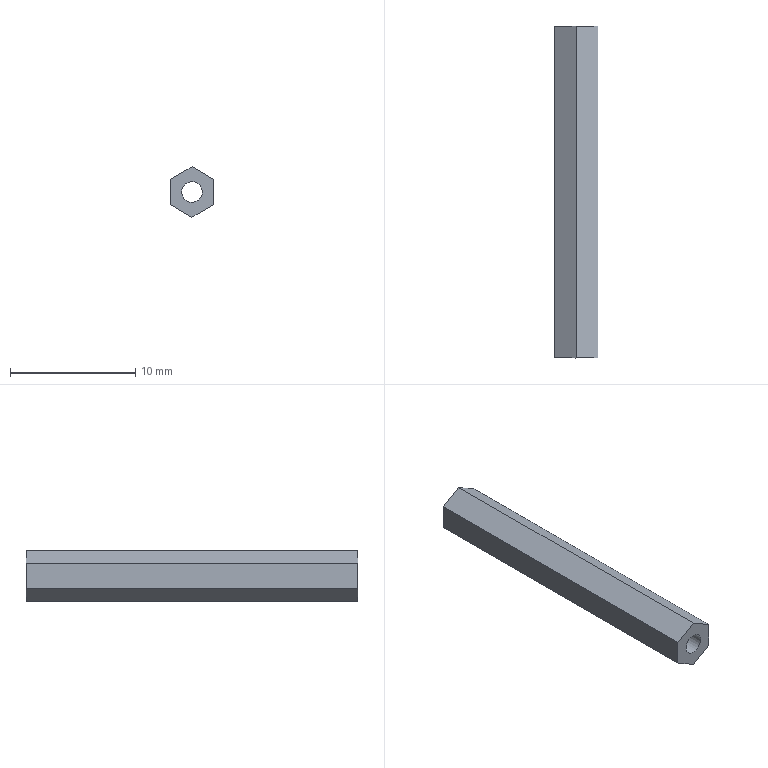Component | NX | 12 | 1 solid | 9 faces | box 3.51 x 26.5 x 4.04 mm | volume 224 mm3 | plane 8 | cylinder 1 | commonest cylinder face diameters 1.65 x1
STEP:
#1=CARTESIAN_POINT('',(0.,0.,0.));
#2=DIRECTION('',(0.,0.,1.));
#3=DIRECTION('',(1.,0.,0.));
#4=AXIS2_PLACEMENT_3D('',#1,#2,#3);
#5=CARTESIAN_POINT('',(-341.815,190.749,-163.207));
#6=VERTEX_POINT('',#5);
#7=CARTESIAN_POINT('',(-341.815,164.249,-163.207));
#8=VERTEX_POINT('',#7);
#9=CARTESIAN_POINT('',(-341.815,164.249,-163.207));
#10=DIRECTION('',(0.,-1.,0.));
#11=VECTOR('',#10,1.);
#12=LINE('',#9,#11);
#13=CARTESIAN_POINT('',(-340.071,164.249,-164.228));
#14=DIRECTION('',(-0.5052,0.,-0.863));
#15=DIRECTION('',(-0.863,0.,0.5052));
#16=AXIS2_PLACEMENT_3D('',#13,#14,#15);
#17=PLANE('',#16);
#18=CARTESIAN_POINT('',(2.021,0.));
#19=DIRECTION('',(0.,-1.));
#20=VECTOR('',#19,1.);
#21=LINE('',#18,#20);
#22=(GEOMETRIC_REPRESENTATION_CONTEXT(2)PARAMETRIC_REPRESENTATION_CONTEXT()REPRESENTATION_CONTEXT('',''));
#23=DEFINITIONAL_REPRESENTATION('',(#21),#22);
#24=PCURVE('',#17,#23);
#25=CARTESIAN_POINT('',(-341.815,164.249,-163.207));
#26=DIRECTION('',(0.4948,0.,-0.869));
#27=DIRECTION('',(0.,-1.,0.));
#28=AXIS2_PLACEMENT_3D('',#25,#26,#27);
#29=PLANE('',#28);
#30=CARTESIAN_POINT('',(0.,0.));
#31=DIRECTION('',(1.,0.));
#32=VECTOR('',#31,1.);
#33=LINE('',#30,#32);
#34=(GEOMETRIC_REPRESENTATION_CONTEXT(2)PARAMETRIC_REPRESENTATION_CONTEXT()REPRESENTATION_CONTEXT('',''));
#35=DEFINITIONAL_REPRESENTATION('',(#33),#34);
#36=PCURVE('',#29,#35);
#37=SURFACE_CURVE('',#12,(#24,#36),.PCURVE_S1.);
#38=EDGE_CURVE('',#6,#8,#37,.T.);
#39=ORIENTED_EDGE('',*,*,#38,.T.);
#40=CARTESIAN_POINT('',(-340.071,164.249,-164.228));
#41=VERTEX_POINT('',#40);
#42=CARTESIAN_POINT('',(-340.071,164.249,-164.228));
#43=DIRECTION('',(-0.863,0.,0.5052));
#44=VECTOR('',#43,1.);
#45=LINE('',#42,#44);
#46=CARTESIAN_POINT('',(0.,0.));
#47=DIRECTION('',(1.,0.));
#48=VECTOR('',#47,1.);
#49=LINE('',#46,#48);
#50=(GEOMETRIC_REPRESENTATION_CONTEXT(2)PARAMETRIC_REPRESENTATION_CONTEXT()REPRESENTATION_CONTEXT('',''));
#51=DEFINITIONAL_REPRESENTATION('',(#49),#50);
#52=PCURVE('',#17,#51);
#53=CARTESIAN_POINT('',(-341.827,164.249,-165.227));
#54=DIRECTION('',(0.,-1.,0.));
#55=DIRECTION('',(-0.869,0.,-0.4948));
#56=AXIS2_PLACEMENT_3D('',#53,#54,#55);
#57=PLANE('',#56);
#58=CARTESIAN_POINT('',(-2.021,-0.));
#59=DIRECTION('',(0.5,-0.866));
#60=VECTOR('',#59,1.);
#61=LINE('',#58,#60);
#62=(GEOMETRIC_REPRESENTATION_CONTEXT(2)PARAMETRIC_REPRESENTATION_CONTEXT()REPRESENTATION_CONTEXT('',''));
#63=DEFINITIONAL_REPRESENTATION('',(#61),#62);
#64=PCURVE('',#57,#63);
#65=SURFACE_CURVE('',#45,(#52,#64),.PCURVE_S1.);
#66=EDGE_CURVE('',#41,#8,#65,.T.);
#67=ORIENTED_EDGE('',*,*,#66,.F.);
#68=CARTESIAN_POINT('',(-340.071,190.749,-164.228));
#69=VERTEX_POINT('',#68);
#70=CARTESIAN_POINT('',(-340.071,164.249,-164.228));
#71=DIRECTION('',(0.,1.,0.));
#72=VECTOR('',#71,1.);
#73=LINE('',#70,#72);
#74=CARTESIAN_POINT('',(0.,0.));
#75=DIRECTION('',(0.,1.));
#76=VECTOR('',#75,1.);
#77=LINE('',#74,#76);
#78=(GEOMETRIC_REPRESENTATION_CONTEXT(2)PARAMETRIC_REPRESENTATION_CONTEXT()REPRESENTATION_CONTEXT('',''));
#79=DEFINITIONAL_REPRESENTATION('',(#77),#78);
#80=PCURVE('',#17,#79);
#81=CARTESIAN_POINT('',(-340.083,164.249,-166.248));
#82=DIRECTION('',(-1.,0.,0.005967));
#83=DIRECTION('',(0.005967,0.,1.));
#84=AXIS2_PLACEMENT_3D('',#81,#82,#83);
#85=PLANE('',#84);
#86=CARTESIAN_POINT('',(2.021,0.));
#87=DIRECTION('',(0.,1.));
#88=VECTOR('',#87,1.);
#89=LINE('',#86,#88);
#90=(GEOMETRIC_REPRESENTATION_CONTEXT(2)PARAMETRIC_REPRESENTATION_CONTEXT()REPRESENTATION_CONTEXT('',''));
#91=DEFINITIONAL_REPRESENTATION('',(#89),#90);
#92=PCURVE('',#85,#91);
#93=SURFACE_CURVE('',#73,(#80,#92),.PCURVE_S1.);
#94=EDGE_CURVE('',#41,#69,#93,.T.);
#95=ORIENTED_EDGE('',*,*,#94,.T.);
#96=CARTESIAN_POINT('',(-340.071,190.749,-164.228));
#97=DIRECTION('',(-0.863,0.,0.5052));
#98=VECTOR('',#97,1.);
#99=LINE('',#96,#98);
#100=CARTESIAN_POINT('',(0.,26.5));
#101=DIRECTION('',(1.,0.));
#102=VECTOR('',#101,1.);
#103=LINE('',#100,#102);
#104=(GEOMETRIC_REPRESENTATION_CONTEXT(2)PARAMETRIC_REPRESENTATION_CONTEXT()REPRESENTATION_CONTEXT('',''));
#105=DEFINITIONAL_REPRESENTATION('',(#103),#104);
#106=PCURVE('',#17,#105);
#107=CARTESIAN_POINT('',(-341.827,190.749,-165.227));
#108=DIRECTION('',(0.,-1.,0.));
#109=DIRECTION('',(-0.869,0.,-0.4948));
#110=AXIS2_PLACEMENT_3D('',#107,#108,#109);
#111=PLANE('',#110);
#112=CARTESIAN_POINT('',(-2.021,-0.));
#113=DIRECTION('',(0.5,-0.866));
#114=VECTOR('',#113,1.);
#115=LINE('',#112,#114);
#116=(GEOMETRIC_REPRESENTATION_CONTEXT(2)PARAMETRIC_REPRESENTATION_CONTEXT()REPRESENTATION_CONTEXT('',''));
#117=DEFINITIONAL_REPRESENTATION('',(#115),#116);
#118=PCURVE('',#111,#117);
#119=SURFACE_CURVE('',#99,(#106,#118),.PCURVE_S1.);
#120=EDGE_CURVE('',#69,#6,#119,.T.);
#121=ORIENTED_EDGE('',*,*,#120,.T.);
#122=EDGE_LOOP('',(#39,#67,#95,#121));
#123=FACE_BOUND('',#122,.T.);
#124=ADVANCED_FACE('',(#123),#17,.F.);
#125=CARTESIAN_POINT('',(-343.571,190.749,-164.207));
#126=VERTEX_POINT('',#125);
#127=CARTESIAN_POINT('',(-343.571,164.249,-164.207));
#128=VERTEX_POINT('',#127);
#129=CARTESIAN_POINT('',(-343.571,164.249,-164.207));
#130=DIRECTION('',(0.,-1.,0.));
#131=VECTOR('',#130,1.);
#132=LINE('',#129,#131);
#133=CARTESIAN_POINT('',(0.,2.021));
#134=DIRECTION('',(1.,0.));
#135=VECTOR('',#134,1.);
#136=LINE('',#133,#135);
#137=(GEOMETRIC_REPRESENTATION_CONTEXT(2)PARAMETRIC_REPRESENTATION_CONTEXT()REPRESENTATION_CONTEXT('',''));
#138=DEFINITIONAL_REPRESENTATION('',(#136),#137);
#139=PCURVE('',#29,#138);
#140=CARTESIAN_POINT('',(-343.571,164.249,-164.207));
#141=DIRECTION('',(1.,0.,-0.005967));
#142=DIRECTION('',(-0.005967,0.,-1.));
#143=AXIS2_PLACEMENT_3D('',#140,#141,#142);
#144=PLANE('',#143);
#145=CARTESIAN_POINT('',(0.,0.));
#146=DIRECTION('',(0.,-1.));
#147=VECTOR('',#146,1.);
#148=LINE('',#145,#147);
#149=(GEOMETRIC_REPRESENTATION_CONTEXT(2)PARAMETRIC_REPRESENTATION_CONTEXT()REPRESENTATION_CONTEXT('',''));
#150=DEFINITIONAL_REPRESENTATION('',(#148),#149);
#151=PCURVE('',#144,#150);
#152=SURFACE_CURVE('',#132,(#139,#151),.PCURVE_S1.);
#153=EDGE_CURVE('',#126,#128,#152,.T.);
#154=ORIENTED_EDGE('',*,*,#153,.T.);
#155=CARTESIAN_POINT('',(-342.693,164.249,-163.707));
#156=DIRECTION('',(-0.869,0.,-0.4948));
#157=VECTOR('',#156,1.);
#158=LINE('',#155,#157);
#159=CARTESIAN_POINT('',(0.,1.01));
#160=DIRECTION('',(0.,1.));
#161=VECTOR('',#160,1.);
#162=LINE('',#159,#161);
#163=(GEOMETRIC_REPRESENTATION_CONTEXT(2)PARAMETRIC_REPRESENTATION_CONTEXT()REPRESENTATION_CONTEXT('',''));
#164=DEFINITIONAL_REPRESENTATION('',(#162),#163);
#165=PCURVE('',#29,#164);
#166=CARTESIAN_POINT('',(-0.,-1.75));
#167=DIRECTION('',(1.,0.));
#168=VECTOR('',#167,1.);
#169=LINE('',#166,#168);
#170=(GEOMETRIC_REPRESENTATION_CONTEXT(2)PARAMETRIC_REPRESENTATION_CONTEXT()REPRESENTATION_CONTEXT('',''));
#171=DEFINITIONAL_REPRESENTATION('',(#169),#170);
#172=PCURVE('',#57,#171);
#173=SURFACE_CURVE('',#158,(#165,#172),.PCURVE_S1.);
#174=EDGE_CURVE('',#8,#128,#173,.T.);
#175=ORIENTED_EDGE('',*,*,#174,.F.);
#176=ORIENTED_EDGE('',*,*,#38,.F.);
#177=CARTESIAN_POINT('',(-342.693,190.749,-163.707));
#178=DIRECTION('',(-0.869,0.,-0.4948));
#179=VECTOR('',#178,1.);
#180=LINE('',#177,#179);
#181=CARTESIAN_POINT('',(-26.5,1.01));
#182=DIRECTION('',(0.,1.));
#183=VECTOR('',#182,1.);
#184=LINE('',#181,#183);
#185=(GEOMETRIC_REPRESENTATION_CONTEXT(2)PARAMETRIC_REPRESENTATION_CONTEXT()REPRESENTATION_CONTEXT('',''));
#186=DEFINITIONAL_REPRESENTATION('',(#184),#185);
#187=PCURVE('',#29,#186);
#188=CARTESIAN_POINT('',(-0.,-1.75));
#189=DIRECTION('',(1.,0.));
#190=VECTOR('',#189,1.);
#191=LINE('',#188,#190);
#192=(GEOMETRIC_REPRESENTATION_CONTEXT(2)PARAMETRIC_REPRESENTATION_CONTEXT()REPRESENTATION_CONTEXT('',''));
#193=DEFINITIONAL_REPRESENTATION('',(#191),#192);
#194=PCURVE('',#111,#193);
#195=SURFACE_CURVE('',#180,(#187,#194),.PCURVE_S1.);
#196=EDGE_CURVE('',#6,#126,#195,.T.);
#197=ORIENTED_EDGE('',*,*,#196,.T.);
#198=EDGE_LOOP('',(#154,#175,#176,#197));
#199=FACE_BOUND('',#198,.T.);
#200=ADVANCED_FACE('',(#199),#29,.F.);
#201=CARTESIAN_POINT('',(-343.583,190.749,-166.227));
#202=VERTEX_POINT('',#201);
#203=CARTESIAN_POINT('',(-343.583,164.249,-166.227));
#204=VERTEX_POINT('',#203);
#205=CARTESIAN_POINT('',(-343.583,164.249,-166.227));
#206=DIRECTION('',(0.,-1.,0.));
#207=VECTOR('',#206,1.);
#208=LINE('',#205,#207);
#209=CARTESIAN_POINT('',(2.021,0.));
#210=DIRECTION('',(0.,-1.));
#211=VECTOR('',#210,1.);
#212=LINE('',#209,#211);
#213=(GEOMETRIC_REPRESENTATION_CONTEXT(2)PARAMETRIC_REPRESENTATION_CONTEXT()REPRESENTATION_CONTEXT('',''));
#214=DEFINITIONAL_REPRESENTATION('',(#212),#213);
#215=PCURVE('',#144,#214);
#216=CARTESIAN_POINT('',(-343.583,164.249,-166.227));
#217=DIRECTION('',(0.5052,0.,0.863));
#218=DIRECTION('',(0.863,0.,-0.5052));
#219=AXIS2_PLACEMENT_3D('',#216,#217,#218);
#220=PLANE('',#219);
#221=CARTESIAN_POINT('',(0.,0.));
#222=DIRECTION('',(0.,-1.));
#223=VECTOR('',#222,1.);
#224=LINE('',#221,#223);
#225=(GEOMETRIC_REPRESENTATION_CONTEXT(2)PARAMETRIC_REPRESENTATION_CONTEXT()REPRESENTATION_CONTEXT('',''));
#226=DEFINITIONAL_REPRESENTATION('',(#224),#225);
#227=PCURVE('',#220,#226);
#228=SURFACE_CURVE('',#208,(#215,#227),.PCURVE_S1.);
#229=EDGE_CURVE('',#202,#204,#228,.T.);
#230=ORIENTED_EDGE('',*,*,#229,.T.);
#231=CARTESIAN_POINT('',(-343.571,164.249,-164.207));
#232=DIRECTION('',(-0.005967,0.,-1.));
#233=VECTOR('',#232,1.);
#234=LINE('',#231,#233);
#235=CARTESIAN_POINT('',(0.,0.));
#236=DIRECTION('',(1.,0.));
#237=VECTOR('',#236,1.);
#238=LINE('',#235,#237);
#239=(GEOMETRIC_REPRESENTATION_CONTEXT(2)PARAMETRIC_REPRESENTATION_CONTEXT()REPRESENTATION_CONTEXT('',''));
#240=DEFINITIONAL_REPRESENTATION('',(#238),#239);
#241=PCURVE('',#144,#240);
#242=CARTESIAN_POINT('',(1.01,-1.75));
#243=DIRECTION('',(0.5,0.866));
#244=VECTOR('',#243,1.);
#245=LINE('',#242,#244);
#246=(GEOMETRIC_REPRESENTATION_CONTEXT(2)PARAMETRIC_REPRESENTATION_CONTEXT()REPRESENTATION_CONTEXT('',''));
#247=DEFINITIONAL_REPRESENTATION('',(#245),#246);
#248=PCURVE('',#57,#247);
#249=SURFACE_CURVE('',#234,(#241,#248),.PCURVE_S1.);
#250=EDGE_CURVE('',#128,#204,#249,.T.);
#251=ORIENTED_EDGE('',*,*,#250,.F.);
#252=ORIENTED_EDGE('',*,*,#153,.F.);
#253=CARTESIAN_POINT('',(-343.571,190.749,-164.207));
#254=DIRECTION('',(-0.005967,0.,-1.));
#255=VECTOR('',#254,1.);
#256=LINE('',#253,#255);
#257=CARTESIAN_POINT('',(0.,26.5));
#258=DIRECTION('',(1.,0.));
#259=VECTOR('',#258,1.);
#260=LINE('',#257,#259);
#261=(GEOMETRIC_REPRESENTATION_CONTEXT(2)PARAMETRIC_REPRESENTATION_CONTEXT()REPRESENTATION_CONTEXT('',''));
#262=DEFINITIONAL_REPRESENTATION('',(#260),#261);
#263=PCURVE('',#144,#262);
#264=CARTESIAN_POINT('',(1.01,-1.75));
#265=DIRECTION('',(0.5,0.866));
#266=VECTOR('',#265,1.);
#267=LINE('',#264,#266);
#268=(GEOMETRIC_REPRESENTATION_CONTEXT(2)PARAMETRIC_REPRESENTATION_CONTEXT()REPRESENTATION_CONTEXT('',''));
#269=DEFINITIONAL_REPRESENTATION('',(#267),#268);
#270=PCURVE('',#111,#269);
#271=SURFACE_CURVE('',#256,(#263,#270),.PCURVE_S1.);
#272=EDGE_CURVE('',#126,#202,#271,.T.);
#273=ORIENTED_EDGE('',*,*,#272,.T.);
#274=EDGE_LOOP('',(#230,#251,#252,#273));
#275=FACE_BOUND('',#274,.T.);
#276=ADVANCED_FACE('',(#275),#144,.F.);
#277=CARTESIAN_POINT('',(-341.839,190.749,-167.248));
#278=VERTEX_POINT('',#277);
#279=CARTESIAN_POINT('',(-341.839,164.249,-167.248));
#280=VERTEX_POINT('',#279);
#281=CARTESIAN_POINT('',(-341.839,164.249,-167.248));
#282=DIRECTION('',(0.,-1.,0.));
#283=VECTOR('',#282,1.);
#284=LINE('',#281,#283);
#285=CARTESIAN_POINT('',(2.021,0.));
#286=DIRECTION('',(0.,-1.));
#287=VECTOR('',#286,1.);
#288=LINE('',#285,#287);
#289=(GEOMETRIC_REPRESENTATION_CONTEXT(2)PARAMETRIC_REPRESENTATION_CONTEXT()REPRESENTATION_CONTEXT('',''));
#290=DEFINITIONAL_REPRESENTATION('',(#288),#289);
#291=PCURVE('',#220,#290);
#292=CARTESIAN_POINT('',(-341.839,164.249,-167.248));
#293=DIRECTION('',(-0.4948,0.,0.869));
#294=DIRECTION('',(0.869,0.,0.4948));
#295=AXIS2_PLACEMENT_3D('',#292,#293,#294);
#296=PLANE('',#295);
#297=CARTESIAN_POINT('',(0.,0.));
#298=DIRECTION('',(0.,-1.));
#299=VECTOR('',#298,1.);
#300=LINE('',#297,#299);
#301=(GEOMETRIC_REPRESENTATION_CONTEXT(2)PARAMETRIC_REPRESENTATION_CONTEXT()REPRESENTATION_CONTEXT('',''));
#302=DEFINITIONAL_REPRESENTATION('',(#300),#301);
#303=PCURVE('',#296,#302);
#304=SURFACE_CURVE('',#284,(#291,#303),.PCURVE_S1.);
#305=EDGE_CURVE('',#278,#280,#304,.T.);
#306=ORIENTED_EDGE('',*,*,#305,.T.);
#307=CARTESIAN_POINT('',(-343.583,164.249,-166.227));
#308=DIRECTION('',(0.863,0.,-0.5052));
#309=VECTOR('',#308,1.);
#310=LINE('',#307,#309);
#311=CARTESIAN_POINT('',(0.,0.));
#312=DIRECTION('',(1.,0.));
#313=VECTOR('',#312,1.);
#314=LINE('',#311,#313);
#315=(GEOMETRIC_REPRESENTATION_CONTEXT(2)PARAMETRIC_REPRESENTATION_CONTEXT()REPRESENTATION_CONTEXT('',''));
#316=DEFINITIONAL_REPRESENTATION('',(#314),#315);
#317=PCURVE('',#220,#316);
#318=CARTESIAN_POINT('',(2.021,-0.));
#319=DIRECTION('',(-0.5,0.866));
#320=VECTOR('',#319,1.);
#321=LINE('',#318,#320);
#322=(GEOMETRIC_REPRESENTATION_CONTEXT(2)PARAMETRIC_REPRESENTATION_CONTEXT()REPRESENTATION_CONTEXT('',''));
#323=DEFINITIONAL_REPRESENTATION('',(#321),#322);
#324=PCURVE('',#57,#323);
#325=SURFACE_CURVE('',#310,(#317,#324),.PCURVE_S1.);
#326=EDGE_CURVE('',#204,#280,#325,.T.);
#327=ORIENTED_EDGE('',*,*,#326,.F.);
#328=ORIENTED_EDGE('',*,*,#229,.F.);
#329=CARTESIAN_POINT('',(-343.583,190.749,-166.227));
#330=DIRECTION('',(0.863,0.,-0.5052));
#331=VECTOR('',#330,1.);
#332=LINE('',#329,#331);
#333=CARTESIAN_POINT('',(0.,26.5));
#334=DIRECTION('',(1.,0.));
#335=VECTOR('',#334,1.);
#336=LINE('',#333,#335);
#337=(GEOMETRIC_REPRESENTATION_CONTEXT(2)PARAMETRIC_REPRESENTATION_CONTEXT()REPRESENTATION_CONTEXT('',''));
#338=DEFINITIONAL_REPRESENTATION('',(#336),#337);
#339=PCURVE('',#220,#338);
#340=CARTESIAN_POINT('',(2.021,-0.));
#341=DIRECTION('',(-0.5,0.866));
#342=VECTOR('',#341,1.);
#343=LINE('',#340,#342);
#344=(GEOMETRIC_REPRESENTATION_CONTEXT(2)PARAMETRIC_REPRESENTATION_CONTEXT()REPRESENTATION_CONTEXT('',''));
#345=DEFINITIONAL_REPRESENTATION('',(#343),#344);
#346=PCURVE('',#111,#345);
#347=SURFACE_CURVE('',#332,(#339,#346),.PCURVE_S1.);
#348=EDGE_CURVE('',#202,#278,#347,.T.);
#349=ORIENTED_EDGE('',*,*,#348,.T.);
#350=EDGE_LOOP('',(#306,#327,#328,#349));
#351=FACE_BOUND('',#350,.T.);
#352=ADVANCED_FACE('',(#351),#220,.F.);
#353=CARTESIAN_POINT('',(-340.083,190.749,-166.248));
#354=VERTEX_POINT('',#353);
#355=CARTESIAN_POINT('',(-340.083,164.249,-166.248));
#356=VERTEX_POINT('',#355);
#357=CARTESIAN_POINT('',(-340.083,164.249,-166.248));
#358=DIRECTION('',(0.,-1.,0.));
#359=VECTOR('',#358,1.);
#360=LINE('',#357,#359);
#361=CARTESIAN_POINT('',(2.021,0.));
#362=DIRECTION('',(0.,-1.));
#363=VECTOR('',#362,1.);
#364=LINE('',#361,#363);
#365=(GEOMETRIC_REPRESENTATION_CONTEXT(2)PARAMETRIC_REPRESENTATION_CONTEXT()REPRESENTATION_CONTEXT('',''));
#366=DEFINITIONAL_REPRESENTATION('',(#364),#365);
#367=PCURVE('',#296,#366);
#368=CARTESIAN_POINT('',(0.,0.));
#369=DIRECTION('',(0.,-1.));
#370=VECTOR('',#369,1.);
#371=LINE('',#368,#370);
#372=(GEOMETRIC_REPRESENTATION_CONTEXT(2)PARAMETRIC_REPRESENTATION_CONTEXT()REPRESENTATION_CONTEXT('',''));
#373=DEFINITIONAL_REPRESENTATION('',(#371),#372);
#374=PCURVE('',#85,#373);
#375=SURFACE_CURVE('',#360,(#367,#374),.PCURVE_S1.);
#376=EDGE_CURVE('',#354,#356,#375,.T.);
#377=ORIENTED_EDGE('',*,*,#376,.T.);
#378=CARTESIAN_POINT('',(-340.961,164.249,-166.748));
#379=DIRECTION('',(0.869,0.,0.4948));
#380=VECTOR('',#379,1.);
#381=LINE('',#378,#380);
#382=CARTESIAN_POINT('',(1.01,0.));
#383=DIRECTION('',(1.,0.));
#384=VECTOR('',#383,1.);
#385=LINE('',#382,#384);
#386=(GEOMETRIC_REPRESENTATION_CONTEXT(2)PARAMETRIC_REPRESENTATION_CONTEXT()REPRESENTATION_CONTEXT('',''));
#387=DEFINITIONAL_REPRESENTATION('',(#385),#386);
#388=PCURVE('',#296,#387);
#389=CARTESIAN_POINT('',(-0.,1.75));
#390=DIRECTION('',(-1.,0.));
#391=VECTOR('',#390,1.);
#392=LINE('',#389,#391);
#393=(GEOMETRIC_REPRESENTATION_CONTEXT(2)PARAMETRIC_REPRESENTATION_CONTEXT()REPRESENTATION_CONTEXT('',''));
#394=DEFINITIONAL_REPRESENTATION('',(#392),#393);
#395=PCURVE('',#57,#394);
#396=SURFACE_CURVE('',#381,(#388,#395),.PCURVE_S1.);
#397=EDGE_CURVE('',#280,#356,#396,.T.);
#398=ORIENTED_EDGE('',*,*,#397,.F.);
#399=ORIENTED_EDGE('',*,*,#305,.F.);
#400=CARTESIAN_POINT('',(-340.961,190.749,-166.748));
#401=DIRECTION('',(0.869,0.,0.4948));
#402=VECTOR('',#401,1.);
#403=LINE('',#400,#402);
#404=CARTESIAN_POINT('',(1.01,26.5));
#405=DIRECTION('',(1.,0.));
#406=VECTOR('',#405,1.);
#407=LINE('',#404,#406);
#408=(GEOMETRIC_REPRESENTATION_CONTEXT(2)PARAMETRIC_REPRESENTATION_CONTEXT()REPRESENTATION_CONTEXT('',''));
#409=DEFINITIONAL_REPRESENTATION('',(#407),#408);
#410=PCURVE('',#296,#409);
#411=CARTESIAN_POINT('',(-0.,1.75));
#412=DIRECTION('',(-1.,0.));
#413=VECTOR('',#412,1.);
#414=LINE('',#411,#413);
#415=(GEOMETRIC_REPRESENTATION_CONTEXT(2)PARAMETRIC_REPRESENTATION_CONTEXT()REPRESENTATION_CONTEXT('',''));
#416=DEFINITIONAL_REPRESENTATION('',(#414),#415);
#417=PCURVE('',#111,#416);
#418=SURFACE_CURVE('',#403,(#410,#417),.PCURVE_S1.);
#419=EDGE_CURVE('',#278,#354,#418,.T.);
#420=ORIENTED_EDGE('',*,*,#419,.T.);
#421=EDGE_LOOP('',(#377,#398,#399,#420));
#422=FACE_BOUND('',#421,.T.);
#423=ADVANCED_FACE('',(#422),#296,.F.);
#424=ORIENTED_EDGE('',*,*,#94,.F.);
#425=CARTESIAN_POINT('',(-340.083,164.249,-166.248));
#426=DIRECTION('',(0.005967,0.,1.));
#427=VECTOR('',#426,1.);
#428=LINE('',#425,#427);
#429=CARTESIAN_POINT('',(0.,0.));
#430=DIRECTION('',(1.,0.));
#431=VECTOR('',#430,1.);
#432=LINE('',#429,#431);
#433=(GEOMETRIC_REPRESENTATION_CONTEXT(2)PARAMETRIC_REPRESENTATION_CONTEXT()REPRESENTATION_CONTEXT('',''));
#434=DEFINITIONAL_REPRESENTATION('',(#432),#433);
#435=PCURVE('',#85,#434);
#436=CARTESIAN_POINT('',(-1.01,1.75));
#437=DIRECTION('',(-0.5,-0.866));
#438=VECTOR('',#437,1.);
#439=LINE('',#436,#438);
#440=(GEOMETRIC_REPRESENTATION_CONTEXT(2)PARAMETRIC_REPRESENTATION_CONTEXT()REPRESENTATION_CONTEXT('',''));
#441=DEFINITIONAL_REPRESENTATION('',(#439),#440);
#442=PCURVE('',#57,#441);
#443=SURFACE_CURVE('',#428,(#435,#442),.PCURVE_S1.);
#444=EDGE_CURVE('',#356,#41,#443,.T.);
#445=ORIENTED_EDGE('',*,*,#444,.F.);
#446=ORIENTED_EDGE('',*,*,#376,.F.);
#447=CARTESIAN_POINT('',(-340.083,190.749,-166.248));
#448=DIRECTION('',(0.005967,0.,1.));
#449=VECTOR('',#448,1.);
#450=LINE('',#447,#449);
#451=CARTESIAN_POINT('',(0.,26.5));
#452=DIRECTION('',(1.,0.));
#453=VECTOR('',#452,1.);
#454=LINE('',#451,#453);
#455=(GEOMETRIC_REPRESENTATION_CONTEXT(2)PARAMETRIC_REPRESENTATION_CONTEXT()REPRESENTATION_CONTEXT('',''));
#456=DEFINITIONAL_REPRESENTATION('',(#454),#455);
#457=PCURVE('',#85,#456);
#458=CARTESIAN_POINT('',(-1.01,1.75));
#459=DIRECTION('',(-0.5,-0.866));
#460=VECTOR('',#459,1.);
#461=LINE('',#458,#460);
#462=(GEOMETRIC_REPRESENTATION_CONTEXT(2)PARAMETRIC_REPRESENTATION_CONTEXT()REPRESENTATION_CONTEXT('',''));
#463=DEFINITIONAL_REPRESENTATION('',(#461),#462);
#464=PCURVE('',#111,#463);
#465=SURFACE_CURVE('',#450,(#457,#464),.PCURVE_S1.);
#466=EDGE_CURVE('',#354,#69,#465,.T.);
#467=ORIENTED_EDGE('',*,*,#466,.T.);
#468=EDGE_LOOP('',(#424,#445,#446,#467));
#469=FACE_BOUND('',#468,.T.);
#470=ADVANCED_FACE('',(#469),#85,.F.);
#471=ORIENTED_EDGE('',*,*,#326,.T.);
#472=ORIENTED_EDGE('',*,*,#397,.T.);
#473=ORIENTED_EDGE('',*,*,#444,.T.);
#474=ORIENTED_EDGE('',*,*,#66,.T.);
#475=ORIENTED_EDGE('',*,*,#174,.T.);
#476=ORIENTED_EDGE('',*,*,#250,.T.);
#477=EDGE_LOOP('',(#471,#472,#473,#474,#475,#476));
#478=FACE_BOUND('',#477,.T.);
#479=CARTESIAN_POINT('',(-341.11,164.249,-164.819));
#480=VERTEX_POINT('',#479);
#481=CARTESIAN_POINT('',(-341.827,164.249,-165.227));
#482=DIRECTION('',(0.,1.,0.));
#483=DIRECTION('',(0.869,0.,0.4948));
#484=AXIS2_PLACEMENT_3D('',#481,#482,#483);
#485=CIRCLE('',#484,0.825);
#486=CARTESIAN_POINT('',(-0.825,-0.));
#487=CARTESIAN_POINT('',(-0.825,1.429));
#488=CARTESIAN_POINT('',(0.4125,0.7145));
#489=CARTESIAN_POINT('',(1.65,0.));
#490=CARTESIAN_POINT('',(0.4125,-0.7145));
#491=CARTESIAN_POINT('',(-0.825,-1.429));
#492=CARTESIAN_POINT('',(-0.825,-0.));
#493=(BOUNDED_CURVE()B_SPLINE_CURVE(2,(#486,#487,#488,#489,#490,#491,#492),.UNSPECIFIED.,.T.,.F.)B_SPLINE_CURVE_WITH_KNOTS((1,2,2,2,2,1),(-2.094,0.,2.094,4.189,6.283,8.378),.UNSPECIFIED.)CURVE()GEOMETRIC_REPRESENTATION_ITEM()RATIONAL_B_SPLINE_CURVE((1.,0.5,1.,0.5,1.,0.5,1.))REPRESENTATION_ITEM(''));
#494=(GEOMETRIC_REPRESENTATION_CONTEXT(2)PARAMETRIC_REPRESENTATION_CONTEXT()REPRESENTATION_CONTEXT('',''));
#495=DEFINITIONAL_REPRESENTATION('',(#493),#494);
#496=PCURVE('',#57,#495);
#497=CARTESIAN_POINT('',(-341.827,164.249,-165.227));
#498=DIRECTION('',(0.,-1.,0.));
#499=DIRECTION('',(-0.869,0.,-0.4948));
#500=AXIS2_PLACEMENT_3D('',#497,#498,#499);
#501=CYLINDRICAL_SURFACE('',#500,0.825);
#502=CARTESIAN_POINT('',(9.425,0.));
#503=DIRECTION('',(-1.,0.));
#504=VECTOR('',#503,1.);
#505=LINE('',#502,#504);
#506=(GEOMETRIC_REPRESENTATION_CONTEXT(2)PARAMETRIC_REPRESENTATION_CONTEXT()REPRESENTATION_CONTEXT('',''));
#507=DEFINITIONAL_REPRESENTATION('',(#505),#506);
#508=PCURVE('',#501,#507);
#509=SURFACE_CURVE('',#485,(#496,#508),.PCURVE_S1.);
#510=EDGE_CURVE('',#480,#480,#509,.T.);
#511=ORIENTED_EDGE('',*,*,#510,.T.);
#512=EDGE_LOOP('',(#511));
#513=FACE_BOUND('',#512,.T.);
#514=ADVANCED_FACE('',(#478,#513),#57,.T.);
#515=ORIENTED_EDGE('',*,*,#419,.F.);
#516=ORIENTED_EDGE('',*,*,#348,.F.);
#517=ORIENTED_EDGE('',*,*,#272,.F.);
#518=ORIENTED_EDGE('',*,*,#196,.F.);
#519=ORIENTED_EDGE('',*,*,#120,.F.);
#520=ORIENTED_EDGE('',*,*,#466,.F.);
#521=EDGE_LOOP('',(#515,#516,#517,#518,#519,#520));
#522=FACE_BOUND('',#521,.T.);
#523=CARTESIAN_POINT('',(-341.11,190.749,-164.819));
#524=VERTEX_POINT('',#523);
#525=CARTESIAN_POINT('',(-341.827,190.749,-165.227));
#526=DIRECTION('',(0.,-1.,0.));
#527=DIRECTION('',(0.869,0.,0.4948));
#528=AXIS2_PLACEMENT_3D('',#525,#526,#527);
#529=CIRCLE('',#528,0.825);
#530=CARTESIAN_POINT('',(0.,0.));
#531=DIRECTION('',(-1.,-0.));
#532=AXIS2_PLACEMENT_2D('',#530,#531);
#533=CIRCLE('',#532,0.825);
#534=(GEOMETRIC_REPRESENTATION_CONTEXT(2)PARAMETRIC_REPRESENTATION_CONTEXT()REPRESENTATION_CONTEXT('',''));
#535=DEFINITIONAL_REPRESENTATION('',(#533),#534);
#536=PCURVE('',#111,#535);
#537=CARTESIAN_POINT('',(3.142,-26.5));
#538=DIRECTION('',(1.,0.));
#539=VECTOR('',#538,1.);
#540=LINE('',#537,#539);
#541=(GEOMETRIC_REPRESENTATION_CONTEXT(2)PARAMETRIC_REPRESENTATION_CONTEXT()REPRESENTATION_CONTEXT('',''));
#542=DEFINITIONAL_REPRESENTATION('',(#540),#541);
#543=PCURVE('',#501,#542);
#544=SURFACE_CURVE('',#529,(#536,#543),.PCURVE_S1.);
#545=EDGE_CURVE('',#524,#524,#544,.T.);
#546=ORIENTED_EDGE('',*,*,#545,.T.);
#547=EDGE_LOOP('',(#546));
#548=FACE_BOUND('',#547,.T.);
#549=ADVANCED_FACE('',(#522,#548),#111,.F.);
#550=ORIENTED_EDGE('',*,*,#510,.T.);
#551=CARTESIAN_POINT('',(-341.11,190.749,-164.819));
#552=CARTESIAN_POINT('',(-341.11,164.249,-164.819));
#553=B_SPLINE_CURVE_WITH_KNOTS('',1,(#551,#552),.UNSPECIFIED.,.F.,.F.,(2,2),(-26.5,0.),.PIECEWISE_BEZIER_KNOTS.);
#554=CARTESIAN_POINT('',(3.142,0.));
#555=DIRECTION('',(0.,1.));
#556=VECTOR('',#555,1.);
#557=LINE('',#554,#556);
#558=(GEOMETRIC_REPRESENTATION_CONTEXT(2)PARAMETRIC_REPRESENTATION_CONTEXT()REPRESENTATION_CONTEXT('',''));
#559=DEFINITIONAL_REPRESENTATION('',(#557),#558);
#560=PCURVE('',#501,#559);
#561=CARTESIAN_POINT('',(9.425,0.));
#562=DIRECTION('',(0.,1.));
#563=VECTOR('',#562,1.);
#564=LINE('',#561,#563);
#565=(GEOMETRIC_REPRESENTATION_CONTEXT(2)PARAMETRIC_REPRESENTATION_CONTEXT()REPRESENTATION_CONTEXT('',''));
#566=DEFINITIONAL_REPRESENTATION('',(#564),#565);
#567=PCURVE('',#501,#566);
#568=SEAM_CURVE('',#553,(#560,#567),.PCURVE_S1.);
#569=EDGE_CURVE('',#524,#480,#568,.T.);
#570=ORIENTED_EDGE('',*,*,#569,.F.);
#571=ORIENTED_EDGE('',*,*,#545,.T.);
#572=ORIENTED_EDGE('',*,*,#569,.T.);
#573=EDGE_LOOP('',(#550,#570,#571,#572));
#574=FACE_BOUND('',#573,.F.);
#575=ADVANCED_FACE('',(#574),#501,.F.);
#576=CLOSED_SHELL('',(#124,#200,#276,#352,#423,#470,#514,#549,#575));
#577=MANIFOLD_SOLID_BREP('',#576);
#578=(LENGTH_UNIT()NAMED_UNIT(*)SI_UNIT(.MILLI.,.METRE.));
#579=UNCERTAINTY_MEASURE_WITH_UNIT(LENGTH_MEASURE(0.000001),#578,'','');
#580=(NAMED_UNIT(*)PLANE_ANGLE_UNIT()SI_UNIT($,.RADIAN.));
#581=(NAMED_UNIT(*)SI_UNIT($,.STERADIAN.)SOLID_ANGLE_UNIT());
#582=(GEOMETRIC_REPRESENTATION_CONTEXT(3)GLOBAL_UNCERTAINTY_ASSIGNED_CONTEXT((#579))GLOBAL_UNIT_ASSIGNED_CONTEXT((#578,#580,#581))REPRESENTATION_CONTEXT('',''));
#583=ADVANCED_BREP_SHAPE_REPRESENTATION('',(#4,#577),#582);